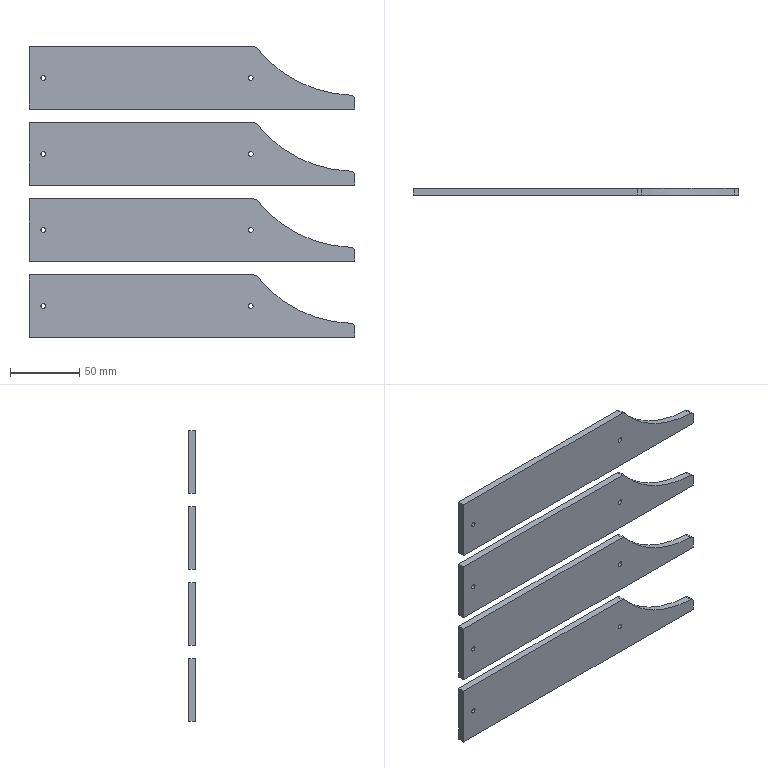CAM job | Mastercam | mm | 4 operations | part box 235 x 5 x 210
1. Contour (Ramp) | 3 - 3 平铣刀
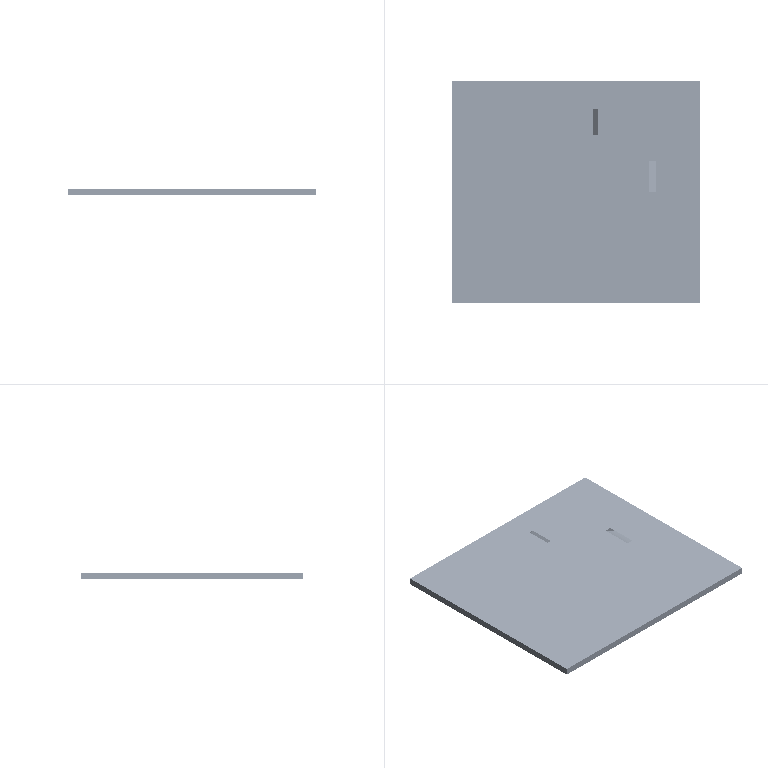2. Contour (2D) | 3 - 3 平铣刀
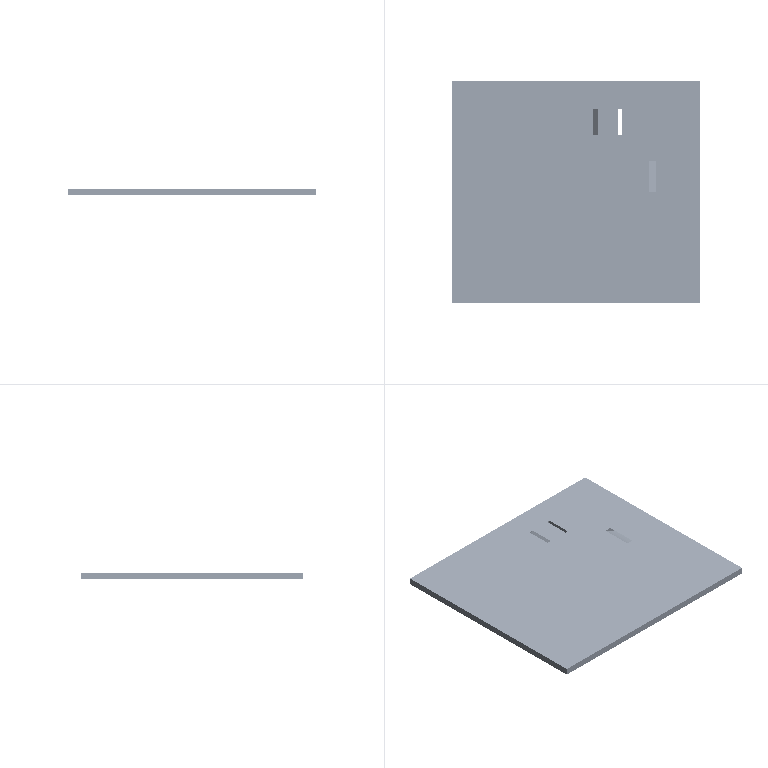3. Drill/Counterbore | 7 - 4 倒角刀
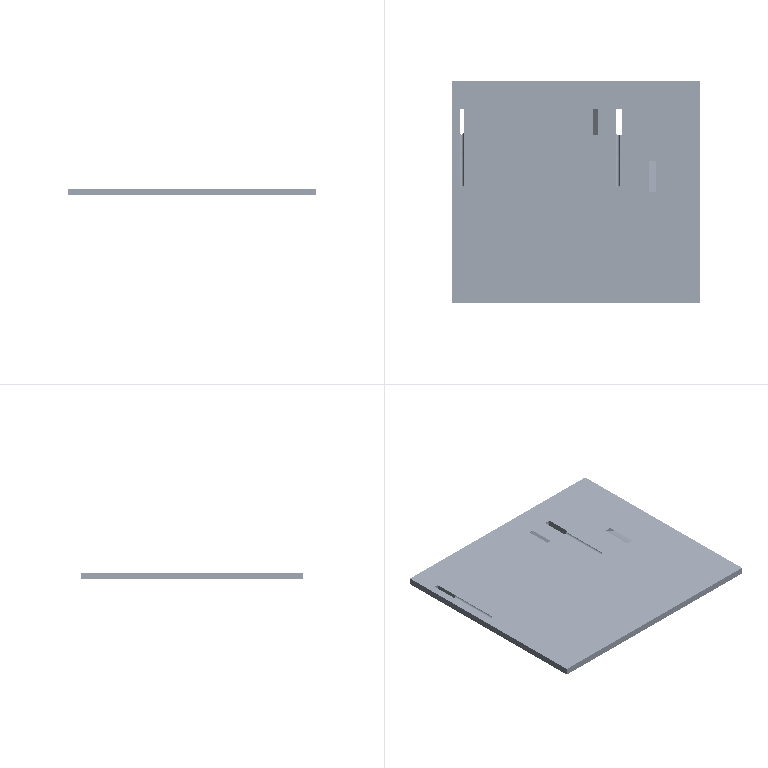4. Contour (2D chamfer) | 7 - 4 倒角刀